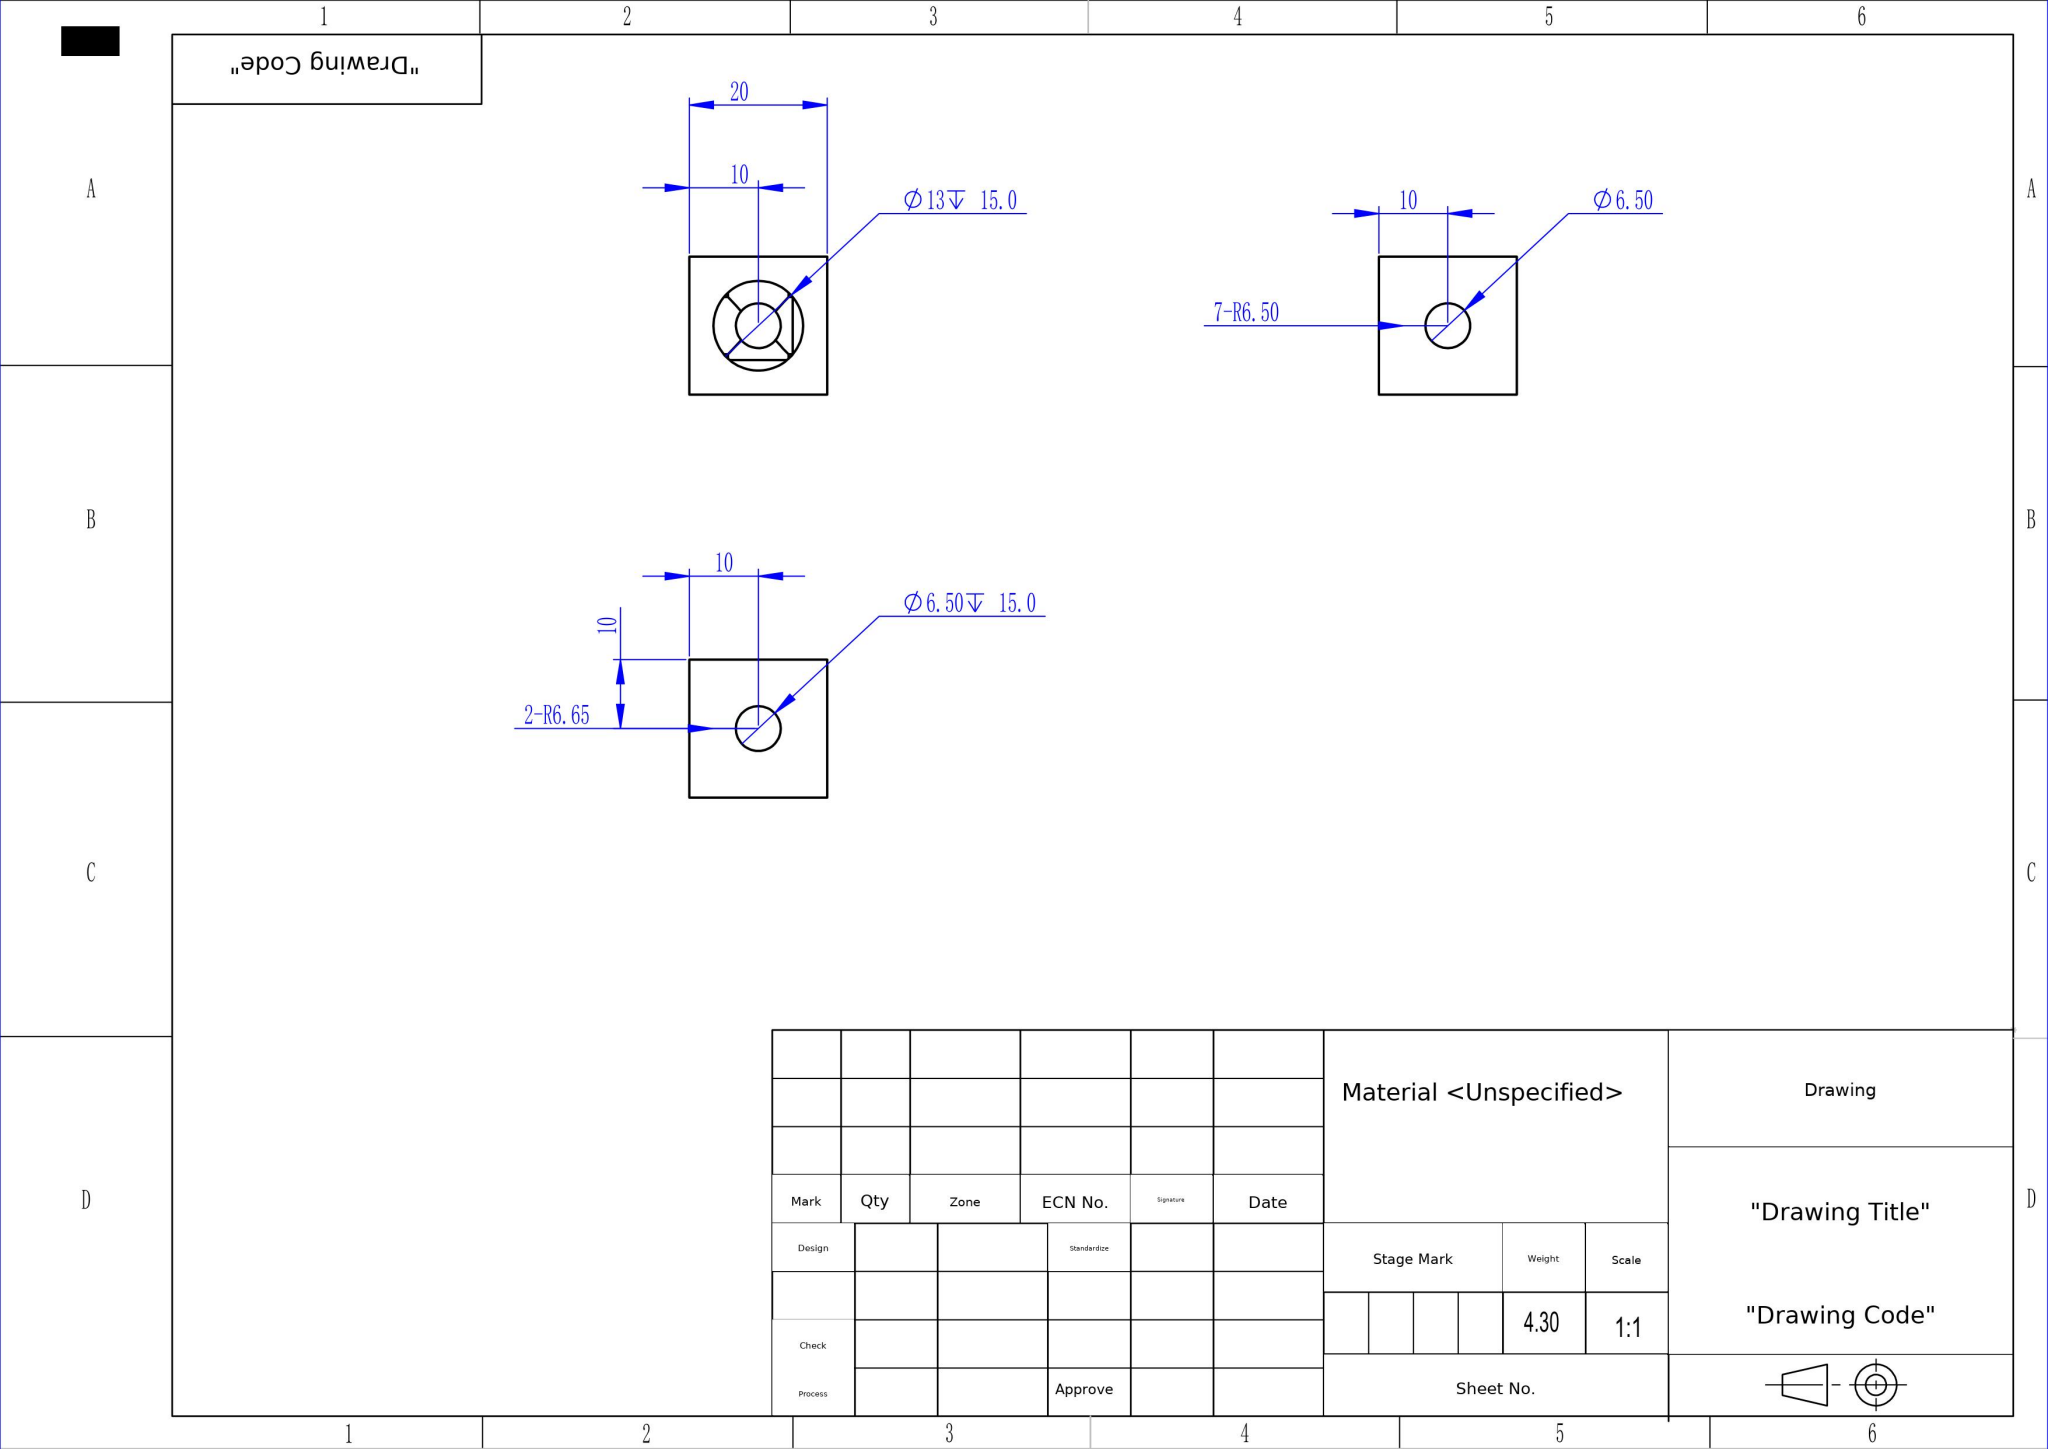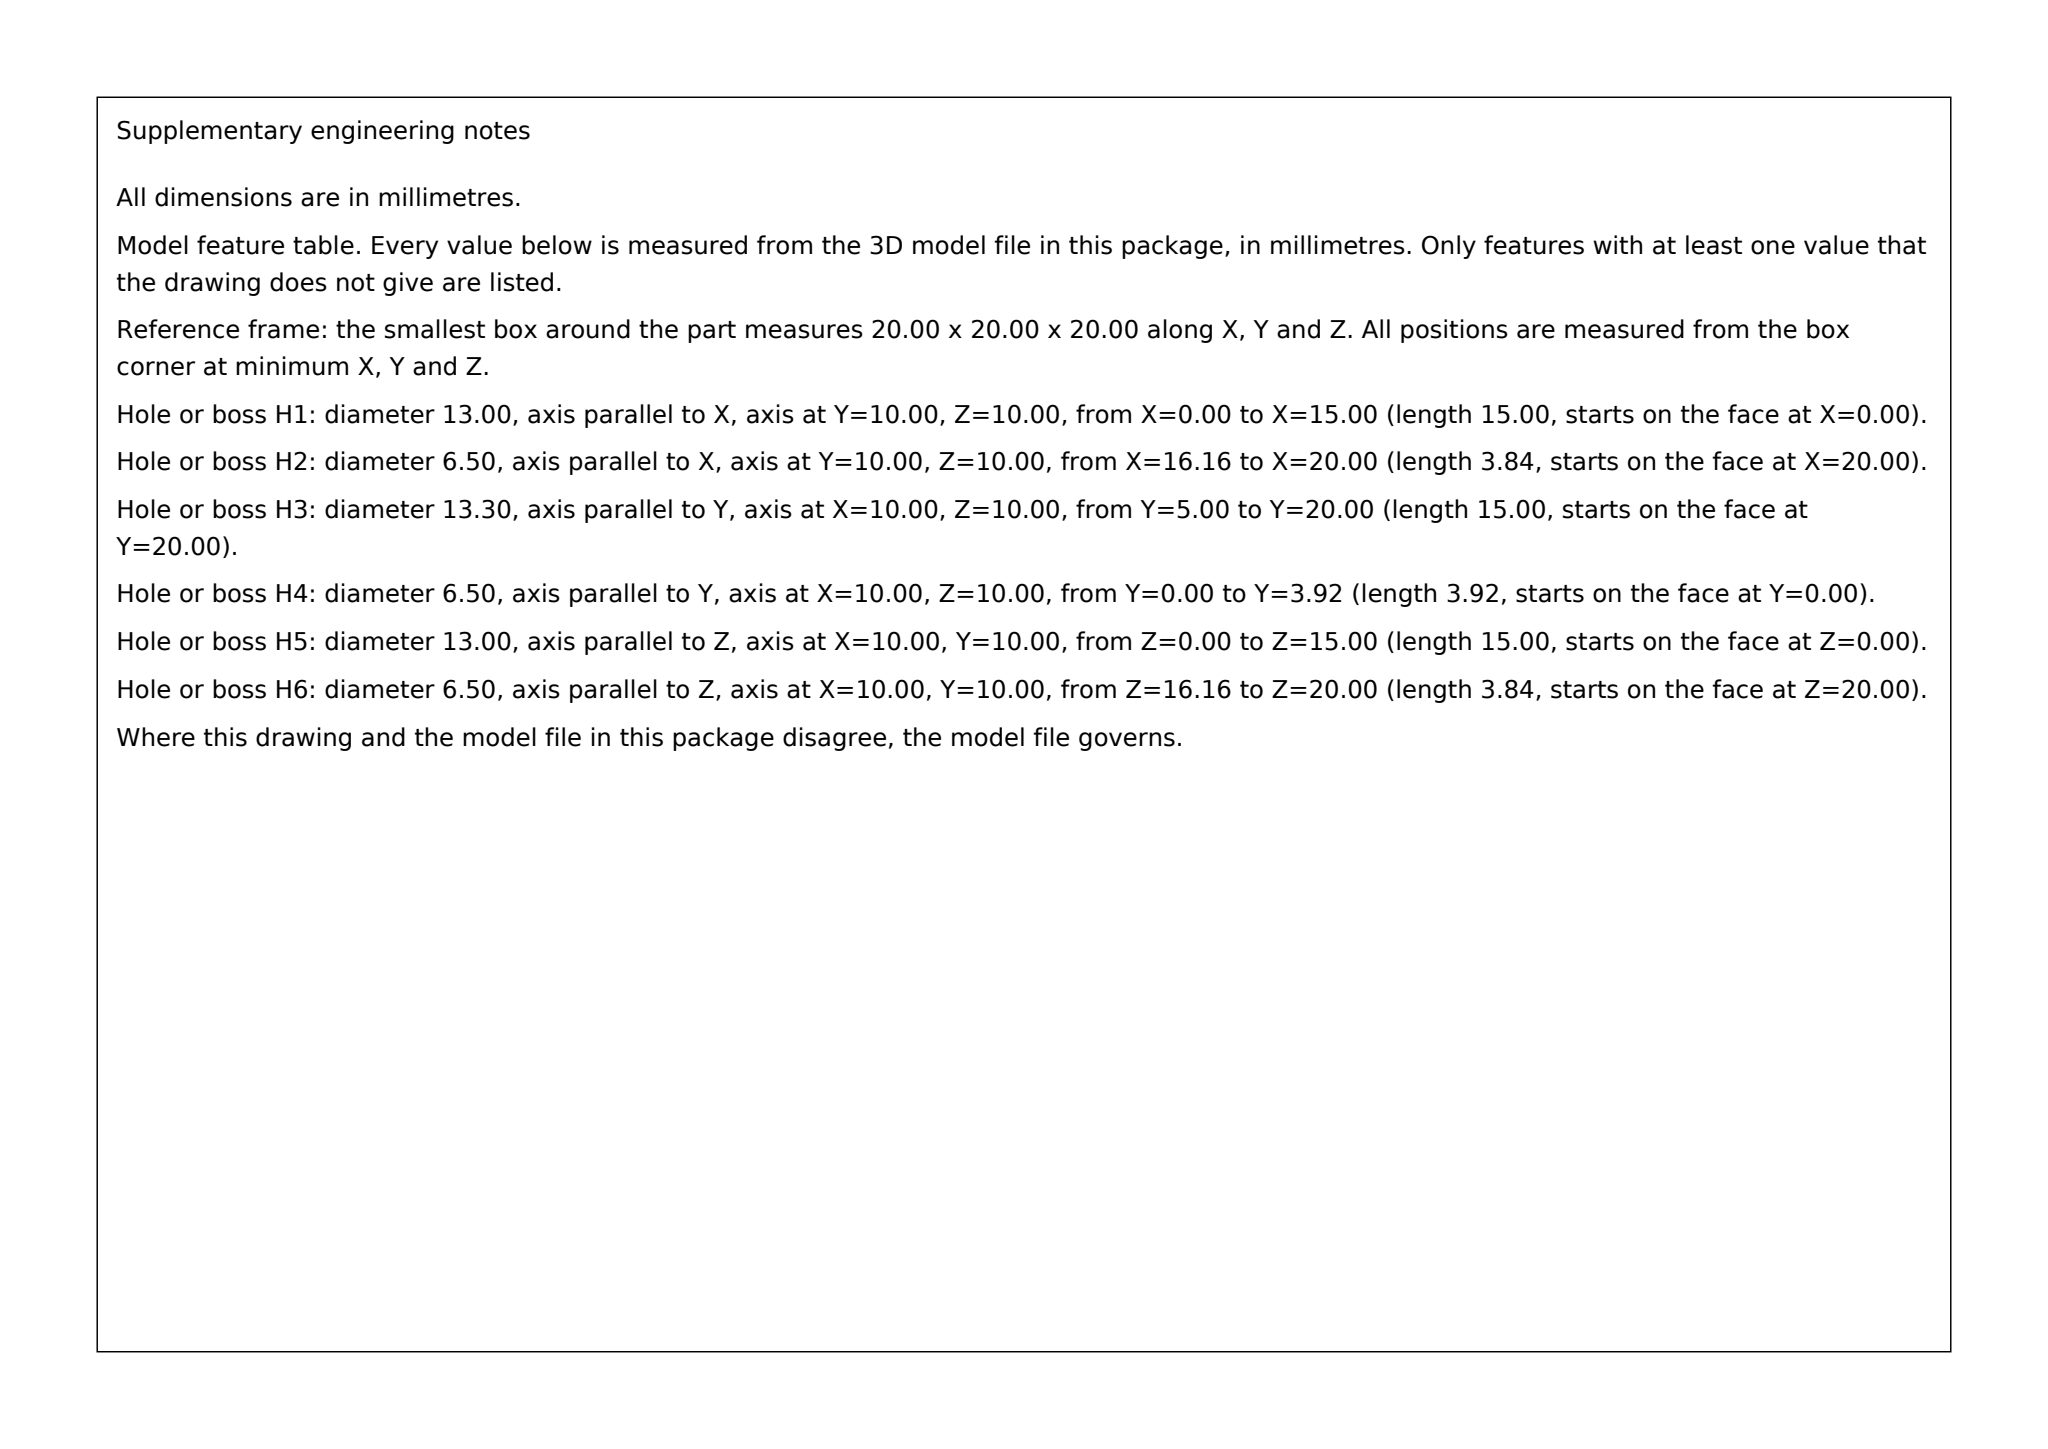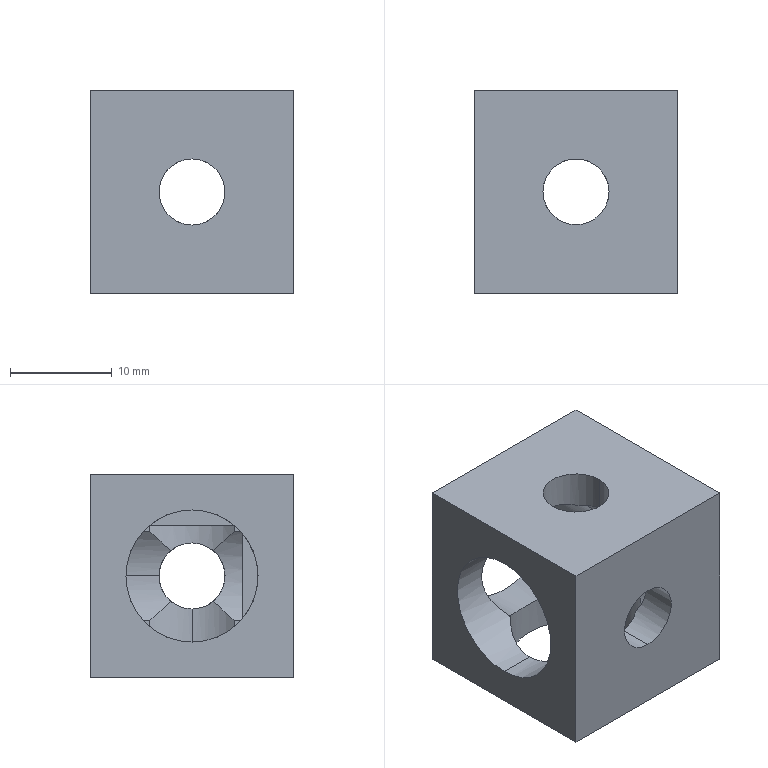Part | SolidWorks | mm | material Unspecified | 1 solid | 47 faces | box 20 x 20 x 20 mm | volume 4298 mm3 | cylinder 27 | plane 20 | commonest cylinder face diameters 13 x17 6.5 x6 13.293 x4
build123d program:
from build123d import *

# Parameters (mm, degrees)
SKETCH1_W               = 20
SKETCH1_H               = 20
BOSS_EXTRUDE1_DEPTH     = 20
CUT_EXTRUDE1_REACH      = 36.641
SKETCH2_R               = 3.25
CUT_EXTRUDE2_REACH      = 36.641
CUT_EXTRUDE2_END_RADIUS = 3.25
SKETCH3_R               = 3.25
SKETCH4_R               = 6.5
CUT_EXTRUDE3_DEPTH      = 15
SKETCH5_R               = 6.5
CUT_EXTRUDE4_DEPTH      = 15
SKETCH6_R               = 6.646
CUT_EXTRUDE5_DEPTH      = 15
SKETCH7_R               = 3.25
CUT_EXTRUDE6_DEPTH      = 15


with BuildPart() as part:
    # Sketch1 → Boss-Extrude1 (new body)
    with BuildSketch(Plane.XY):
        with Locations((-10, 10)):
            Rectangle(SKETCH1_W, SKETCH1_H)
    extrude(amount=BOSS_EXTRUDE1_DEPTH)

    # Sketch2 → Cut-Extrude1 (cut, up to next)
    with BuildSketch(Plane(origin=(0, 0, 0), x_dir=(0, 0, -1), z_dir=(1, 0, 0)), mode=Mode.PRIVATE) as cut_extrude1_sk1:
        with Locations((-10, 10)):
            Circle(SKETCH2_R)
    cut_extrude1_tool1 = extrude(cut_extrude1_sk1.sketch, amount=-CUT_EXTRUDE1_REACH, mode=Mode.PRIVATE) & part.part
    add(cut_extrude1_tool1.solids().sort_by_distance((0, 10, 10))[0], mode=Mode.SUBTRACT)

    # Cut-Extrude2: up to this cylinder (the profile starts outside it)
    cut_extrude2_end = Plane(origin=(-10, 10, 10), z_dir=(1, 0, 0)) * Cylinder(CUT_EXTRUDE2_END_RADIUS, 80.782, mode=Mode.PRIVATE)
    # Sketch3 → Cut-Extrude2 (cut, up to the surface)
    with BuildSketch(Plane.XY.offset(20), mode=Mode.PRIVATE) as cut_extrude2_sk1:
        with Locations((-10, 10)):
            Circle(SKETCH3_R)
    cut_extrude2_tool1 = extrude(cut_extrude2_sk1.sketch, amount=-CUT_EXTRUDE2_REACH, mode=Mode.PRIVATE) - cut_extrude2_end
    add(cut_extrude2_tool1.solids().sort_by_distance((-10, 10, 20))[0], mode=Mode.SUBTRACT)

    # Sketch4 → Cut-Extrude3 (cut)
    with BuildSketch(Plane.ZY.offset(20)):
        with Locations((10, 10)):
            Circle(SKETCH4_R)
    extrude(amount=-CUT_EXTRUDE3_DEPTH, mode=Mode.SUBTRACT)

    # Sketch5 → Cut-Extrude4 (cut)
    with BuildSketch(Plane(origin=(0, 0, 0), x_dir=(-1, 0, 0), z_dir=(0, 0, -1))):
        with Locations((10, 10)):
            Circle(SKETCH5_R)
    extrude(amount=-CUT_EXTRUDE4_DEPTH, mode=Mode.SUBTRACT)

    # Sketch6 → Cut-Extrude5 (cut)
    with BuildSketch(Plane(origin=(0, 20, 0), x_dir=(1, 0, 0), z_dir=(0, 1, 0))):
        with Locations(Location((-10, -10, 0), (0, 0, 180))):
            Circle(SKETCH6_R)
    extrude(amount=-CUT_EXTRUDE5_DEPTH, mode=Mode.SUBTRACT)

    # Sketch7 → Cut-Extrude6 (cut)
    with BuildSketch(Plane.XZ):
        with Locations(Location((-10, 10, 0), (0, 0, 270))):
            Circle(SKETCH7_R)
    extrude(amount=-CUT_EXTRUDE6_DEPTH, mode=Mode.SUBTRACT)


solid = part.part